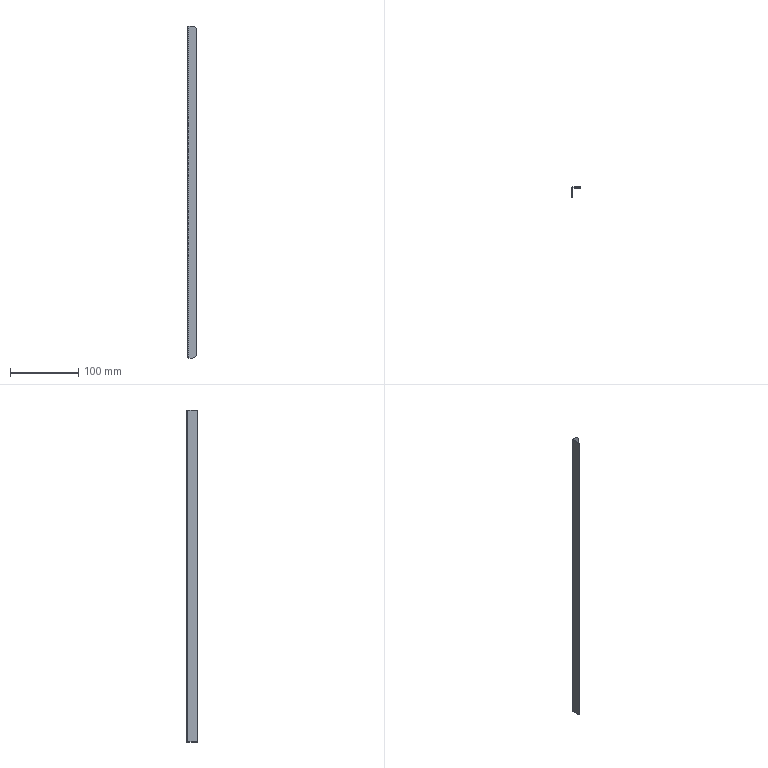Component | SolidWorks | MainBodyWeldment-1_ShelfBeam-1 | 1 solid | 20 faces | box 12 x 15 x 485 mm | volume 18269 mm3 | plane 16 | cylinder 4 | commonest cylinder face diameters 10 x2 3.2 x1 0.2 x1 | material SPCC
STEP:
#1=COLOUR_RGB('',0.7922,0.8196,0.9333);
#2=FILL_AREA_STYLE_COLOUR('',#1);
#3=FILL_AREA_STYLE('',(#2));
#4=SURFACE_STYLE_FILL_AREA(#3);
#5=SURFACE_SIDE_STYLE('',(#4));
#6=SURFACE_STYLE_USAGE(.BOTH.,#5);
#7=PRESENTATION_STYLE_ASSIGNMENT((#6));
#8=CARTESIAN_POINT('',(-7.976,-0.9106,9.291));
#9=VERTEX_POINT('',#8);
#10=CARTESIAN_POINT('',(-7.976,-0.9106,9.284));
#11=VERTEX_POINT('',#10);
#12=CARTESIAN_POINT('',(-7.976,-0.9106,9.291));
#13=DIRECTION('',(0.,0.,-1.));
#14=VECTOR('',#13,39.37);
#15=LINE('',#12,#14);
#16=EDGE_CURVE('',#9,#11,#15,.T.);
#17=ORIENTED_EDGE('',*,*,#16,.T.);
#18=CARTESIAN_POINT('',(-7.984,-0.9106,9.284));
#19=VERTEX_POINT('',#18);
#20=CARTESIAN_POINT('',(-7.925,-0.9106,9.284));
#21=DIRECTION('',(-1.,0.,0.));
#22=VECTOR('',#21,39.37);
#23=LINE('',#20,#22);
#24=EDGE_CURVE('',#11,#19,#23,.T.);
#25=ORIENTED_EDGE('',*,*,#24,.T.);
#26=CARTESIAN_POINT('',(-7.984,-0.9106,-9.795));
#27=VERTEX_POINT('',#26);
#28=CARTESIAN_POINT('',(-7.984,-0.9106,9.291));
#29=DIRECTION('',(0.,0.,-1.));
#30=VECTOR('',#29,39.37);
#31=LINE('',#28,#30);
#32=EDGE_CURVE('',#19,#27,#31,.T.);
#33=ORIENTED_EDGE('',*,*,#32,.T.);
#34=CARTESIAN_POINT('',(-7.976,-0.9106,-9.795));
#35=VERTEX_POINT('',#34);
#36=CARTESIAN_POINT('',(-7.925,-0.9106,-9.795));
#37=DIRECTION('',(1.,0.,0.));
#38=VECTOR('',#37,39.37);
#39=LINE('',#36,#38);
#40=EDGE_CURVE('',#27,#35,#39,.T.);
#41=ORIENTED_EDGE('',*,*,#40,.T.);
#42=CARTESIAN_POINT('',(-7.976,-0.9106,-9.803));
#43=VERTEX_POINT('',#42);
#44=CARTESIAN_POINT('',(-7.976,-0.9106,9.291));
#45=DIRECTION('',(0.,0.,-1.));
#46=VECTOR('',#45,39.37);
#47=LINE('',#44,#46);
#48=EDGE_CURVE('',#35,#43,#47,.T.);
#49=ORIENTED_EDGE('',*,*,#48,.T.);
#50=CARTESIAN_POINT('',(-7.925,-0.9106,-9.803));
#51=VERTEX_POINT('',#50);
#52=CARTESIAN_POINT('',(-7.925,-0.9106,-9.803));
#53=DIRECTION('',(-1.,0.,0.));
#54=VECTOR('',#53,39.37);
#55=LINE('',#52,#54);
#56=EDGE_CURVE('',#51,#43,#55,.T.);
#57=ORIENTED_EDGE('',*,*,#56,.F.);
#58=CARTESIAN_POINT('',(-7.925,-0.9106,9.291));
#59=VERTEX_POINT('',#58);
#60=CARTESIAN_POINT('',(-7.925,-0.9106,9.291));
#61=DIRECTION('',(0.,0.,-1.));
#62=VECTOR('',#61,39.37);
#63=LINE('',#60,#62);
#64=EDGE_CURVE('',#59,#51,#63,.T.);
#65=ORIENTED_EDGE('',*,*,#64,.F.);
#66=CARTESIAN_POINT('',(-7.925,-0.9106,9.291));
#67=DIRECTION('',(-1.,0.,0.));
#68=VECTOR('',#67,39.37);
#69=LINE('',#66,#68);
#70=EDGE_CURVE('',#59,#9,#69,.T.);
#71=ORIENTED_EDGE('',*,*,#70,.T.);
#72=EDGE_LOOP('',(#17,#25,#33,#41,#49,#57,#65,#71));
#73=FACE_OUTER_BOUND('',#72,.T.);
#74=CARTESIAN_POINT('',(-7.925,-0.9106,9.291));
#75=DIRECTION('',(0.,-1.,0.));
#76=DIRECTION('',(0.,0.,-1.));
#77=AXIS2_PLACEMENT_3D('',#74,#75,#76);
#78=PLANE('',#77);
#79=ADVANCED_FACE('',(#73),#78,.T.);
#80=CARTESIAN_POINT('',(-7.976,-0.383,9.291));
#81=VERTEX_POINT('',#80);
#82=CARTESIAN_POINT('',(-7.976,-0.3525,9.291));
#83=VERTEX_POINT('',#82);
#84=CARTESIAN_POINT('',(-7.976,-0.32,9.291));
#85=DIRECTION('',(0.,1.,0.));
#86=VECTOR('',#85,39.37);
#87=LINE('',#84,#86);
#88=EDGE_CURVE('',#81,#83,#87,.T.);
#89=ORIENTED_EDGE('',*,*,#88,.F.);
#90=CARTESIAN_POINT('',(-7.925,-0.383,9.291));
#91=VERTEX_POINT('',#90);
#92=CARTESIAN_POINT('',(-7.925,-0.383,9.291));
#93=DIRECTION('',(-1.,0.,0.));
#94=VECTOR('',#93,39.37);
#95=LINE('',#92,#94);
#96=EDGE_CURVE('',#91,#81,#95,.T.);
#97=ORIENTED_EDGE('',*,*,#96,.F.);
#98=CARTESIAN_POINT('',(-7.921,-0.3791,9.291));
#99=VERTEX_POINT('',#98);
#100=CARTESIAN_POINT('',(-7.921,-0.383,9.291));
#101=DIRECTION('',(0.,0.,-1.));
#102=DIRECTION('',(1.,0.,0.));
#103=AXIS2_PLACEMENT_3D('',#100,#101,#102);
#104=CIRCLE('',#103,0.003937);
#105=EDGE_CURVE('',#91,#99,#104,.T.);
#106=ORIENTED_EDGE('',*,*,#105,.T.);
#107=CARTESIAN_POINT('',(-7.921,-0.32,9.291));
#108=VERTEX_POINT('',#107);
#109=CARTESIAN_POINT('',(-7.921,-0.32,9.291));
#110=DIRECTION('',(0.,-1.,0.));
#111=VECTOR('',#110,39.37);
#112=LINE('',#109,#111);
#113=EDGE_CURVE('',#108,#99,#112,.T.);
#114=ORIENTED_EDGE('',*,*,#113,.F.);
#115=CARTESIAN_POINT('',(-7.921,-0.383,9.291));
#116=DIRECTION('',(0.,0.,-1.));
#117=DIRECTION('',(1.,0.,0.));
#118=AXIS2_PLACEMENT_3D('',#115,#116,#117);
#119=CIRCLE('',#118,0.06299);
#120=EDGE_CURVE('',#83,#108,#119,.T.);
#121=ORIENTED_EDGE('',*,*,#120,.F.);
#122=EDGE_LOOP('',(#89,#97,#106,#114,#121));
#123=FACE_OUTER_BOUND('',#122,.T.);
#124=CARTESIAN_POINT('',(-7.921,-0.32,9.291));
#125=DIRECTION('',(0.,0.,1.));
#126=DIRECTION('',(1.,0.,0.));
#127=AXIS2_PLACEMENT_3D('',#124,#125,#126);
#128=PLANE('',#127);
#129=ADVANCED_FACE('',(#123),#128,.T.);
#130=CARTESIAN_POINT('',(-7.708,-0.3791,9.291));
#131=VERTEX_POINT('',#130);
#132=CARTESIAN_POINT('',(-7.984,-0.3791,9.291));
#133=DIRECTION('',(1.,0.,0.));
#134=VECTOR('',#133,39.37);
#135=LINE('',#132,#134);
#136=EDGE_CURVE('',#99,#131,#135,.T.);
#137=ORIENTED_EDGE('',*,*,#136,.T.);
#138=CARTESIAN_POINT('',(-7.708,-0.32,9.291));
#139=VERTEX_POINT('',#138);
#140=CARTESIAN_POINT('',(-7.708,-0.383,9.291));
#141=DIRECTION('',(0.,1.,0.));
#142=VECTOR('',#141,39.37);
#143=LINE('',#140,#142);
#144=EDGE_CURVE('',#131,#139,#143,.T.);
#145=ORIENTED_EDGE('',*,*,#144,.T.);
#146=CARTESIAN_POINT('',(-7.984,-0.32,9.291));
#147=DIRECTION('',(1.,0.,0.));
#148=VECTOR('',#147,39.37);
#149=LINE('',#146,#148);
#150=EDGE_CURVE('',#108,#139,#149,.T.);
#151=ORIENTED_EDGE('',*,*,#150,.F.);
#152=ORIENTED_EDGE('',*,*,#113,.T.);
#153=EDGE_LOOP('',(#137,#145,#151,#152));
#154=FACE_OUTER_BOUND('',#153,.T.);
#155=CARTESIAN_POINT('',(-7.925,-0.383,9.291));
#156=DIRECTION('',(0.,0.,1.));
#157=DIRECTION('',(1.,0.,0.));
#158=AXIS2_PLACEMENT_3D('',#155,#156,#157);
#159=PLANE('',#158);
#160=ADVANCED_FACE('',(#154),#159,.T.);
#161=CARTESIAN_POINT('',(-7.976,-0.3525,-9.803));
#162=VERTEX_POINT('',#161);
#163=CARTESIAN_POINT('',(-7.976,-0.383,-9.803));
#164=VERTEX_POINT('',#163);
#165=CARTESIAN_POINT('',(-7.976,-0.383,-9.803));
#166=DIRECTION('',(0.,-1.,0.));
#167=VECTOR('',#166,39.37);
#168=LINE('',#165,#167);
#169=EDGE_CURVE('',#162,#164,#168,.T.);
#170=ORIENTED_EDGE('',*,*,#169,.F.);
#171=CARTESIAN_POINT('',(-7.921,-0.32,-9.803));
#172=VERTEX_POINT('',#171);
#173=CARTESIAN_POINT('',(-7.921,-0.383,-9.803));
#174=DIRECTION('',(0.,0.,-1.));
#175=DIRECTION('',(1.,0.,0.));
#176=AXIS2_PLACEMENT_3D('',#173,#174,#175);
#177=CIRCLE('',#176,0.06299);
#178=EDGE_CURVE('',#162,#172,#177,.T.);
#179=ORIENTED_EDGE('',*,*,#178,.T.);
#180=CARTESIAN_POINT('',(-7.921,-0.3791,-9.803));
#181=VERTEX_POINT('',#180);
#182=CARTESIAN_POINT('',(-7.921,-0.3791,-9.803));
#183=DIRECTION('',(0.,1.,0.));
#184=VECTOR('',#183,39.37);
#185=LINE('',#182,#184);
#186=EDGE_CURVE('',#181,#172,#185,.T.);
#187=ORIENTED_EDGE('',*,*,#186,.F.);
#188=CARTESIAN_POINT('',(-7.925,-0.383,-9.803));
#189=VERTEX_POINT('',#188);
#190=CARTESIAN_POINT('',(-7.921,-0.383,-9.803));
#191=DIRECTION('',(0.,0.,-1.));
#192=DIRECTION('',(1.,0.,0.));
#193=AXIS2_PLACEMENT_3D('',#190,#191,#192);
#194=CIRCLE('',#193,0.003937);
#195=EDGE_CURVE('',#189,#181,#194,.T.);
#196=ORIENTED_EDGE('',*,*,#195,.F.);
#197=CARTESIAN_POINT('',(-7.984,-0.383,-9.803));
#198=DIRECTION('',(1.,0.,0.));
#199=VECTOR('',#198,39.37);
#200=LINE('',#197,#199);
#201=EDGE_CURVE('',#164,#189,#200,.T.);
#202=ORIENTED_EDGE('',*,*,#201,.F.);
#203=EDGE_LOOP('',(#170,#179,#187,#196,#202));
#204=FACE_OUTER_BOUND('',#203,.T.);
#205=CARTESIAN_POINT('',(-7.984,-0.383,-9.803));
#206=DIRECTION('',(0.,0.,-1.));
#207=DIRECTION('',(-1.,0.,0.));
#208=AXIS2_PLACEMENT_3D('',#205,#206,#207);
#209=PLANE('',#208);
#210=ADVANCED_FACE('',(#204),#209,.T.);
#211=CARTESIAN_POINT('',(-7.976,-0.3791,-9.803));
#212=DIRECTION('',(0.,-1.,0.));
#213=VECTOR('',#212,39.37);
#214=LINE('',#211,#213);
#215=EDGE_CURVE('',#164,#43,#214,.T.);
#216=ORIENTED_EDGE('',*,*,#215,.F.);
#217=ORIENTED_EDGE('',*,*,#201,.T.);
#218=CARTESIAN_POINT('',(-7.925,-0.9106,-9.803));
#219=DIRECTION('',(0.,1.,0.));
#220=VECTOR('',#219,39.37);
#221=LINE('',#218,#220);
#222=EDGE_CURVE('',#51,#189,#221,.T.);
#223=ORIENTED_EDGE('',*,*,#222,.F.);
#224=ORIENTED_EDGE('',*,*,#56,.T.);
#225=EDGE_LOOP('',(#216,#217,#223,#224));
#226=FACE_OUTER_BOUND('',#225,.T.);
#227=CARTESIAN_POINT('',(-7.921,-0.3791,-9.803));
#228=DIRECTION('',(0.,0.,-1.));
#229=DIRECTION('',(-1.,0.,0.));
#230=AXIS2_PLACEMENT_3D('',#227,#228,#229);
#231=PLANE('',#230);
#232=ADVANCED_FACE('',(#226),#231,.T.);
#233=CARTESIAN_POINT('',(-7.511,-0.3791,9.095));
#234=VERTEX_POINT('',#233);
#235=CARTESIAN_POINT('',(-7.511,-0.3791,-9.606));
#236=VERTEX_POINT('',#235);
#237=CARTESIAN_POINT('',(-7.511,-0.3791,9.291));
#238=DIRECTION('',(0.,0.,-1.));
#239=VECTOR('',#238,39.37);
#240=LINE('',#237,#239);
#241=EDGE_CURVE('',#234,#236,#240,.T.);
#242=ORIENTED_EDGE('',*,*,#241,.F.);
#243=CARTESIAN_POINT('',(-7.708,-0.3791,9.095));
#244=DIRECTION('',(0.,-1.,0.));
#245=DIRECTION('',(0.,0.,1.));
#246=AXIS2_PLACEMENT_3D('',#243,#244,#245);
#247=CIRCLE('',#246,0.1969);
#248=EDGE_CURVE('',#234,#131,#247,.T.);
#249=ORIENTED_EDGE('',*,*,#248,.T.);
#250=ORIENTED_EDGE('',*,*,#136,.F.);
#251=CARTESIAN_POINT('',(-7.921,-0.3791,9.291));
#252=DIRECTION('',(0.,0.,-1.));
#253=VECTOR('',#252,39.37);
#254=LINE('',#251,#253);
#255=EDGE_CURVE('',#99,#181,#254,.T.);
#256=ORIENTED_EDGE('',*,*,#255,.T.);
#257=CARTESIAN_POINT('',(-7.708,-0.3791,-9.803));
#258=VERTEX_POINT('',#257);
#259=CARTESIAN_POINT('',(-7.984,-0.3791,-9.803));
#260=DIRECTION('',(1.,0.,0.));
#261=VECTOR('',#260,39.37);
#262=LINE('',#259,#261);
#263=EDGE_CURVE('',#181,#258,#262,.T.);
#264=ORIENTED_EDGE('',*,*,#263,.T.);
#265=CARTESIAN_POINT('',(-7.708,-0.3791,-9.606));
#266=DIRECTION('',(0.,-1.,0.));
#267=DIRECTION('',(0.,0.,1.));
#268=AXIS2_PLACEMENT_3D('',#265,#266,#267);
#269=CIRCLE('',#268,0.1969);
#270=EDGE_CURVE('',#258,#236,#269,.T.);
#271=ORIENTED_EDGE('',*,*,#270,.T.);
#272=EDGE_LOOP('',(#242,#249,#250,#256,#264,#271));
#273=FACE_OUTER_BOUND('',#272,.T.);
#274=CARTESIAN_POINT('',(-7.984,-0.3791,9.291));
#275=DIRECTION('',(0.,1.,0.));
#276=DIRECTION('',(0.,0.,1.));
#277=AXIS2_PLACEMENT_3D('',#274,#275,#276);
#278=PLANE('',#277);
#279=ADVANCED_FACE('',(#273),#278,.F.);
#280=CARTESIAN_POINT('',(-7.511,-0.32,9.095));
#281=VERTEX_POINT('',#280);
#282=CARTESIAN_POINT('',(-7.511,-0.32,-9.606));
#283=VERTEX_POINT('',#282);
#284=CARTESIAN_POINT('',(-7.511,-0.32,9.291));
#285=DIRECTION('',(0.,0.,-1.));
#286=VECTOR('',#285,39.37);
#287=LINE('',#284,#286);
#288=EDGE_CURVE('',#281,#283,#287,.T.);
#289=ORIENTED_EDGE('',*,*,#288,.F.);
#290=CARTESIAN_POINT('',(-7.511,-0.32,9.095));
#291=DIRECTION('',(0.,-1.,0.));
#292=VECTOR('',#291,39.37);
#293=LINE('',#290,#292);
#294=EDGE_CURVE('',#281,#234,#293,.T.);
#295=ORIENTED_EDGE('',*,*,#294,.T.);
#296=ORIENTED_EDGE('',*,*,#241,.T.);
#297=CARTESIAN_POINT('',(-7.511,-0.32,-9.606));
#298=DIRECTION('',(0.,1.,0.));
#299=VECTOR('',#298,39.37);
#300=LINE('',#297,#299);
#301=EDGE_CURVE('',#236,#283,#300,.T.);
#302=ORIENTED_EDGE('',*,*,#301,.T.);
#303=EDGE_LOOP('',(#289,#295,#296,#302));
#304=FACE_OUTER_BOUND('',#303,.T.);
#305=CARTESIAN_POINT('',(-7.511,-0.32,9.291));
#306=DIRECTION('',(1.,0.,0.));
#307=DIRECTION('',(0.,0.,-1.));
#308=AXIS2_PLACEMENT_3D('',#305,#306,#307);
#309=PLANE('',#308);
#310=ADVANCED_FACE('',(#304),#309,.T.);
#311=ORIENTED_EDGE('',*,*,#150,.T.);
#312=CARTESIAN_POINT('',(-7.708,-0.32,9.095));
#313=DIRECTION('',(0.,1.,0.));
#314=DIRECTION('',(0.,0.,1.));
#315=AXIS2_PLACEMENT_3D('',#312,#313,#314);
#316=CIRCLE('',#315,0.1969);
#317=EDGE_CURVE('',#139,#281,#316,.T.);
#318=ORIENTED_EDGE('',*,*,#317,.T.);
#319=ORIENTED_EDGE('',*,*,#288,.T.);
#320=CARTESIAN_POINT('',(-7.708,-0.32,-9.803));
#321=VERTEX_POINT('',#320);
#322=CARTESIAN_POINT('',(-7.708,-0.32,-9.606));
#323=DIRECTION('',(0.,1.,0.));
#324=DIRECTION('',(0.,0.,1.));
#325=AXIS2_PLACEMENT_3D('',#322,#323,#324);
#326=CIRCLE('',#325,0.1969);
#327=EDGE_CURVE('',#283,#321,#326,.T.);
#328=ORIENTED_EDGE('',*,*,#327,.T.);
#329=CARTESIAN_POINT('',(-7.984,-0.32,-9.803));
#330=DIRECTION('',(1.,0.,0.));
#331=VECTOR('',#330,39.37);
#332=LINE('',#329,#331);
#333=EDGE_CURVE('',#172,#321,#332,.T.);
#334=ORIENTED_EDGE('',*,*,#333,.F.);
#335=CARTESIAN_POINT('',(-7.921,-0.32,9.291));
#336=DIRECTION('',(0.,0.,-1.));
#337=VECTOR('',#336,39.37);
#338=LINE('',#335,#337);
#339=EDGE_CURVE('',#108,#172,#338,.T.);
#340=ORIENTED_EDGE('',*,*,#339,.F.);
#341=EDGE_LOOP('',(#311,#318,#319,#328,#334,#340));
#342=FACE_OUTER_BOUND('',#341,.T.);
#343=CARTESIAN_POINT('',(-7.984,-0.32,9.291));
#344=DIRECTION('',(0.,1.,0.));
#345=DIRECTION('',(0.,0.,1.));
#346=AXIS2_PLACEMENT_3D('',#343,#344,#345);
#347=PLANE('',#346);
#348=ADVANCED_FACE('',(#342),#347,.T.);
#349=CARTESIAN_POINT('',(-7.976,-0.3525,9.284));
#350=VERTEX_POINT('',#349);
#351=CARTESIAN_POINT('',(-7.984,-0.383,9.284));
#352=VERTEX_POINT('',#351);
#353=CARTESIAN_POINT('',(-7.921,-0.383,9.284));
#354=DIRECTION('',(0.,0.,1.));
#355=DIRECTION('',(-1.,-0.,0.));
#356=AXIS2_PLACEMENT_3D('',#353,#354,#355);
#357=CIRCLE('',#356,0.06299);
#358=EDGE_CURVE('',#350,#352,#357,.T.);
#359=ORIENTED_EDGE('',*,*,#358,.F.);
#360=CARTESIAN_POINT('',(-7.976,-0.3525,9.291));
#361=DIRECTION('',(0.,0.,-1.));
#362=VECTOR('',#361,39.37);
#363=LINE('',#360,#362);
#364=EDGE_CURVE('',#83,#350,#363,.T.);
#365=ORIENTED_EDGE('',*,*,#364,.F.);
#366=ORIENTED_EDGE('',*,*,#120,.T.);
#367=ORIENTED_EDGE('',*,*,#339,.T.);
#368=ORIENTED_EDGE('',*,*,#178,.F.);
#369=CARTESIAN_POINT('',(-7.976,-0.3525,-9.795));
#370=VERTEX_POINT('',#369);
#371=CARTESIAN_POINT('',(-7.976,-0.3525,9.291));
#372=DIRECTION('',(0.,0.,-1.));
#373=VECTOR('',#372,39.37);
#374=LINE('',#371,#373);
#375=EDGE_CURVE('',#370,#162,#374,.T.);
#376=ORIENTED_EDGE('',*,*,#375,.F.);
#377=CARTESIAN_POINT('',(-7.984,-0.383,-9.795));
#378=VERTEX_POINT('',#377);
#379=CARTESIAN_POINT('',(-7.921,-0.383,-9.795));
#380=DIRECTION('',(0.,0.,-1.));
#381=DIRECTION('',(1.,-0.,0.));
#382=AXIS2_PLACEMENT_3D('',#379,#380,#381);
#383=CIRCLE('',#382,0.06299);
#384=EDGE_CURVE('',#378,#370,#383,.T.);
#385=ORIENTED_EDGE('',*,*,#384,.F.);
#386=CARTESIAN_POINT('',(-7.984,-0.383,9.291));
#387=DIRECTION('',(0.,0.,-1.));
#388=VECTOR('',#387,39.37);
#389=LINE('',#386,#388);
#390=EDGE_CURVE('',#352,#378,#389,.T.);
#391=ORIENTED_EDGE('',*,*,#390,.F.);
#392=EDGE_LOOP('',(#359,#365,#366,#367,#368,#376,#385,#391));
#393=FACE_OUTER_BOUND('',#392,.T.);
#394=CARTESIAN_POINT('',(-7.921,-0.383,9.291));
#395=DIRECTION('',(0.,0.,-1.));
#396=DIRECTION('',(-1.,0.,0.));
#397=AXIS2_PLACEMENT_3D('',#394,#395,#396);
#398=CYLINDRICAL_SURFACE('',#397,0.06299);
#399=ADVANCED_FACE('',(#393),#398,.T.);
#400=CARTESIAN_POINT('',(-7.984,-0.9106,9.284));
#401=DIRECTION('',(0.,-1.,0.));
#402=VECTOR('',#401,39.37);
#403=LINE('',#400,#402);
#404=EDGE_CURVE('',#352,#19,#403,.T.);
#405=ORIENTED_EDGE('',*,*,#404,.F.);
#406=ORIENTED_EDGE('',*,*,#390,.T.);
#407=CARTESIAN_POINT('',(-7.984,-0.9106,-9.795));
#408=DIRECTION('',(0.,1.,0.));
#409=VECTOR('',#408,39.37);
#410=LINE('',#407,#409);
#411=EDGE_CURVE('',#27,#378,#410,.T.);
#412=ORIENTED_EDGE('',*,*,#411,.F.);
#413=ORIENTED_EDGE('',*,*,#32,.F.);
#414=EDGE_LOOP('',(#405,#406,#412,#413));
#415=FACE_OUTER_BOUND('',#414,.T.);
#416=CARTESIAN_POINT('',(-7.984,-0.9106,9.291));
#417=DIRECTION('',(-1.,0.,0.));
#418=DIRECTION('',(0.,0.,1.));
#419=AXIS2_PLACEMENT_3D('',#416,#417,#418);
#420=PLANE('',#419);
#421=ADVANCED_FACE('',(#415),#420,.T.);
#422=ORIENTED_EDGE('',*,*,#222,.T.);
#423=CARTESIAN_POINT('',(-7.925,-0.383,9.291));
#424=DIRECTION('',(0.,0.,-1.));
#425=VECTOR('',#424,39.37);
#426=LINE('',#423,#425);
#427=EDGE_CURVE('',#91,#189,#426,.T.);
#428=ORIENTED_EDGE('',*,*,#427,.F.);
#429=CARTESIAN_POINT('',(-7.925,-0.9106,9.291));
#430=DIRECTION('',(0.,1.,0.));
#431=VECTOR('',#430,39.37);
#432=LINE('',#429,#431);
#433=EDGE_CURVE('',#59,#91,#432,.T.);
#434=ORIENTED_EDGE('',*,*,#433,.F.);
#435=ORIENTED_EDGE('',*,*,#64,.T.);
#436=EDGE_LOOP('',(#422,#428,#434,#435));
#437=FACE_OUTER_BOUND('',#436,.T.);
#438=CARTESIAN_POINT('',(-7.925,-0.9106,9.291));
#439=DIRECTION('',(-1.,0.,0.));
#440=DIRECTION('',(0.,0.,1.));
#441=AXIS2_PLACEMENT_3D('',#438,#439,#440);
#442=PLANE('',#441);
#443=ADVANCED_FACE('',(#437),#442,.F.);
#444=ORIENTED_EDGE('',*,*,#195,.T.);
#445=ORIENTED_EDGE('',*,*,#255,.F.);
#446=ORIENTED_EDGE('',*,*,#105,.F.);
#447=ORIENTED_EDGE('',*,*,#427,.T.);
#448=EDGE_LOOP('',(#444,#445,#446,#447));
#449=FACE_OUTER_BOUND('',#448,.T.);
#450=CARTESIAN_POINT('',(-7.921,-0.383,9.291));
#451=DIRECTION('',(0.,0.,-1.));
#452=DIRECTION('',(-1.,0.,0.));
#453=AXIS2_PLACEMENT_3D('',#450,#451,#452);
#454=CYLINDRICAL_SURFACE('',#453,0.003937);
#455=ADVANCED_FACE('',(#449),#454,.F.);
#456=CARTESIAN_POINT('',(-7.976,-0.383,9.291));
#457=DIRECTION('',(0.,1.,0.));
#458=VECTOR('',#457,39.37);
#459=LINE('',#456,#458);
#460=EDGE_CURVE('',#9,#81,#459,.T.);
#461=ORIENTED_EDGE('',*,*,#460,.F.);
#462=ORIENTED_EDGE('',*,*,#70,.F.);
#463=ORIENTED_EDGE('',*,*,#433,.T.);
#464=ORIENTED_EDGE('',*,*,#96,.T.);
#465=EDGE_LOOP('',(#461,#462,#463,#464));
#466=FACE_OUTER_BOUND('',#465,.T.);
#467=CARTESIAN_POINT('',(-7.921,-0.383,9.291));
#468=DIRECTION('',(0.,0.,1.));
#469=DIRECTION('',(1.,0.,0.));
#470=AXIS2_PLACEMENT_3D('',#467,#468,#469);
#471=PLANE('',#470);
#472=ADVANCED_FACE('',(#466),#471,.T.);
#473=ORIENTED_EDGE('',*,*,#333,.T.);
#474=CARTESIAN_POINT('',(-7.708,-0.3791,-9.803));
#475=DIRECTION('',(0.,-1.,0.));
#476=VECTOR('',#475,39.37);
#477=LINE('',#474,#476);
#478=EDGE_CURVE('',#321,#258,#477,.T.);
#479=ORIENTED_EDGE('',*,*,#478,.T.);
#480=ORIENTED_EDGE('',*,*,#263,.F.);
#481=ORIENTED_EDGE('',*,*,#186,.T.);
#482=EDGE_LOOP('',(#473,#479,#480,#481));
#483=FACE_OUTER_BOUND('',#482,.T.);
#484=CARTESIAN_POINT('',(-7.921,-0.383,-9.803));
#485=DIRECTION('',(0.,0.,1.));
#486=DIRECTION('',(1.,0.,0.));
#487=AXIS2_PLACEMENT_3D('',#484,#485,#486);
#488=PLANE('',#487);
#489=ADVANCED_FACE('',(#483),#488,.F.);
#490=ORIENTED_EDGE('',*,*,#317,.F.);
#491=ORIENTED_EDGE('',*,*,#144,.F.);
#492=ORIENTED_EDGE('',*,*,#248,.F.);
#493=ORIENTED_EDGE('',*,*,#294,.F.);
#494=EDGE_LOOP('',(#490,#491,#492,#493));
#495=FACE_OUTER_BOUND('',#494,.T.);
#496=CARTESIAN_POINT('',(-7.708,-0.32,9.095));
#497=DIRECTION('',(0.,-1.,0.));
#498=DIRECTION('',(0.,0.,-1.));
#499=AXIS2_PLACEMENT_3D('',#496,#497,#498);
#500=CYLINDRICAL_SURFACE('',#499,0.1969);
#501=ADVANCED_FACE('',(#495),#500,.T.);
#502=ORIENTED_EDGE('',*,*,#327,.F.);
#503=ORIENTED_EDGE('',*,*,#301,.F.);
#504=ORIENTED_EDGE('',*,*,#270,.F.);
#505=ORIENTED_EDGE('',*,*,#478,.F.);
#506=EDGE_LOOP('',(#502,#503,#504,#505));
#507=FACE_OUTER_BOUND('',#506,.T.);
#508=CARTESIAN_POINT('',(-7.708,-0.383,-9.606));
#509=DIRECTION('',(0.,1.,0.));
#510=DIRECTION('',(0.,0.,1.));
#511=AXIS2_PLACEMENT_3D('',#508,#509,#510);
#512=CYLINDRICAL_SURFACE('',#511,0.1969);
#513=ADVANCED_FACE('',(#507),#512,.T.);
#514=ORIENTED_EDGE('',*,*,#215,.T.);
#515=ORIENTED_EDGE('',*,*,#48,.F.);
#516=CARTESIAN_POINT('',(-7.976,-0.9106,-9.795));
#517=DIRECTION('',(0.,1.,0.));
#518=VECTOR('',#517,39.37);
#519=LINE('',#516,#518);
#520=EDGE_CURVE('',#35,#370,#519,.T.);
#521=ORIENTED_EDGE('',*,*,#520,.T.);
#522=ORIENTED_EDGE('',*,*,#375,.T.);
#523=ORIENTED_EDGE('',*,*,#169,.T.);
#524=EDGE_LOOP('',(#514,#515,#521,#522,#523));
#525=FACE_OUTER_BOUND('',#524,.T.);
#526=CARTESIAN_POINT('',(-7.976,-0.9106,-9.807));
#527=DIRECTION('',(1.,0.,0.));
#528=DIRECTION('',(0.,0.,-1.));
#529=AXIS2_PLACEMENT_3D('',#526,#527,#528);
#530=PLANE('',#529);
#531=ADVANCED_FACE('',(#525),#530,.F.);
#532=ORIENTED_EDGE('',*,*,#384,.T.);
#533=ORIENTED_EDGE('',*,*,#520,.F.);
#534=ORIENTED_EDGE('',*,*,#40,.F.);
#535=ORIENTED_EDGE('',*,*,#411,.T.);
#536=EDGE_LOOP('',(#532,#533,#534,#535));
#537=FACE_OUTER_BOUND('',#536,.T.);
#538=CARTESIAN_POINT('',(-7.988,-0.9106,-9.795));
#539=DIRECTION('',(0.,0.,1.));
#540=DIRECTION('',(1.,0.,0.));
#541=AXIS2_PLACEMENT_3D('',#538,#539,#540);
#542=PLANE('',#541);
#543=ADVANCED_FACE('',(#537),#542,.F.);
#544=ORIENTED_EDGE('',*,*,#358,.T.);
#545=ORIENTED_EDGE('',*,*,#404,.T.);
#546=ORIENTED_EDGE('',*,*,#24,.F.);
#547=CARTESIAN_POINT('',(-7.976,-0.9106,9.284));
#548=DIRECTION('',(0.,1.,0.));
#549=VECTOR('',#548,39.37);
#550=LINE('',#547,#549);
#551=EDGE_CURVE('',#11,#350,#550,.T.);
#552=ORIENTED_EDGE('',*,*,#551,.T.);
#553=EDGE_LOOP('',(#544,#545,#546,#552));
#554=FACE_OUTER_BOUND('',#553,.T.);
#555=CARTESIAN_POINT('',(-7.988,-0.9106,9.284));
#556=DIRECTION('',(0.,0.,-1.));
#557=DIRECTION('',(-1.,0.,0.));
#558=AXIS2_PLACEMENT_3D('',#555,#556,#557);
#559=PLANE('',#558);
#560=ADVANCED_FACE('',(#554),#559,.F.);
#561=ORIENTED_EDGE('',*,*,#364,.T.);
#562=ORIENTED_EDGE('',*,*,#551,.F.);
#563=ORIENTED_EDGE('',*,*,#16,.F.);
#564=ORIENTED_EDGE('',*,*,#460,.T.);
#565=ORIENTED_EDGE('',*,*,#88,.T.);
#566=EDGE_LOOP('',(#561,#562,#563,#564,#565));
#567=FACE_OUTER_BOUND('',#566,.T.);
#568=CARTESIAN_POINT('',(-7.976,-0.9106,9.284));
#569=DIRECTION('',(1.,0.,0.));
#570=DIRECTION('',(0.,0.,-1.));
#571=AXIS2_PLACEMENT_3D('',#568,#569,#570);
#572=PLANE('',#571);
#573=ADVANCED_FACE('',(#567),#572,.F.);
#574=CLOSED_SHELL('',(#79,#129,#160,#210,#232,#279,#310,#348,#399,#421,#443,#455,#472,#489,#501,#513,#531,#543,#560,#573));
#575=MANIFOLD_SOLID_BREP('',#574);
#576=STYLED_ITEM('',(#7),#575);
#577=PRESENTATION_LAYER_ASSIGNMENT('','',(#576));
#578=(LENGTH_UNIT()NAMED_UNIT(*)SI_UNIT($,.METRE.));
#579=LENGTH_MEASURE_WITH_UNIT(LENGTH_MEASURE(0.0254),#578);
#580=DIMENSIONAL_EXPONENTS(1.,0.,0.,0.,0.,0.,0.);
#581=(CONVERSION_BASED_UNIT('',#579)LENGTH_UNIT()NAMED_UNIT(#580));
#582=UNCERTAINTY_MEASURE_WITH_UNIT(LENGTH_MEASURE(0.00001),#581,'','');
#583=(NAMED_UNIT(*)PLANE_ANGLE_UNIT()SI_UNIT($,.RADIAN.));
#584=(NAMED_UNIT(*)SI_UNIT($,.STERADIAN.)SOLID_ANGLE_UNIT());
#585=(GEOMETRIC_REPRESENTATION_CONTEXT(3)GLOBAL_UNCERTAINTY_ASSIGNED_CONTEXT((#582))GLOBAL_UNIT_ASSIGNED_CONTEXT((#581,#583,#584))REPRESENTATION_CONTEXT('',''));
#586=MECHANICAL_DESIGN_GEOMETRIC_PRESENTATION_REPRESENTATION('',(#576),#585);
#587=CARTESIAN_POINT('',(0.,0.,0.));
#588=DIRECTION('',(0.,0.,1.));
#589=DIRECTION('',(1.,0.,0.));
#590=AXIS2_PLACEMENT_3D('',#587,#588,#589);
#591=(LENGTH_UNIT()NAMED_UNIT(*)SI_UNIT($,.METRE.));
#592=LENGTH_MEASURE_WITH_UNIT(LENGTH_MEASURE(0.0254),#591);
#593=DIMENSIONAL_EXPONENTS(1.,0.,0.,0.,0.,0.,0.);
#594=(CONVERSION_BASED_UNIT('',#592)LENGTH_UNIT()NAMED_UNIT(#593));
#595=UNCERTAINTY_MEASURE_WITH_UNIT(LENGTH_MEASURE(0.00001),#594,'','');
#596=(NAMED_UNIT(*)PLANE_ANGLE_UNIT()SI_UNIT($,.RADIAN.));
#597=(NAMED_UNIT(*)SI_UNIT($,.STERADIAN.)SOLID_ANGLE_UNIT());
#598=(GEOMETRIC_REPRESENTATION_CONTEXT(3)GLOBAL_UNCERTAINTY_ASSIGNED_CONTEXT((#595))GLOBAL_UNIT_ASSIGNED_CONTEXT((#594,#596,#597))REPRESENTATION_CONTEXT('',''));
#599=ADVANCED_BREP_SHAPE_REPRESENTATION('',(#575,#590),#598);